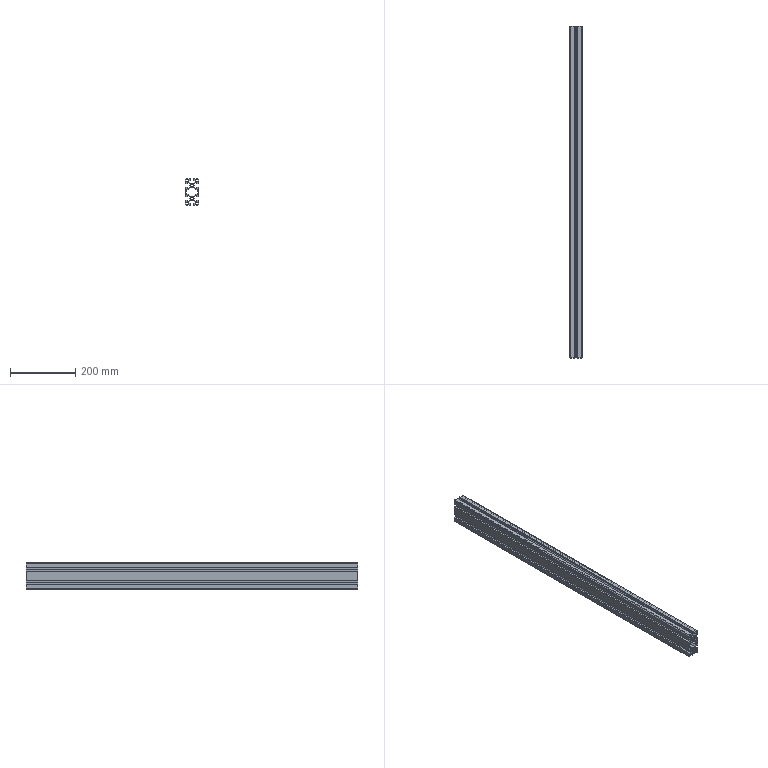Component | SolidWorks | AluminumProfileHFS8-4080Length720-2 | 1 solid | 194 faces | volume 1136294 mm3 | plane 112 | cylinder 82 | commonest cylinder face diameters 2 x36 0.762 x20 0.6 x12 10.5 x10 6 x4 | material 1060 Alloy